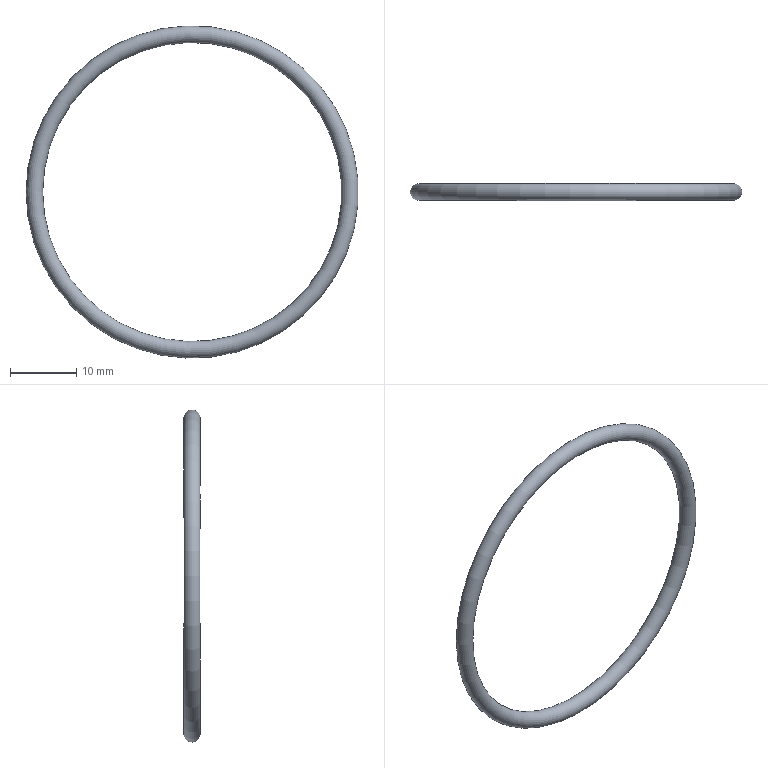Component | NX | O_RING | 1 solid | 1 faces | box 50 x 2.5 x 50 mm | volume 733 mm3 | torus 1
STEP:
#1=CARTESIAN_POINT('',(0.,0.,0.));
#2=DIRECTION('',(0.,0.,1.));
#3=DIRECTION('',(1.,0.,0.));
#4=AXIS2_PLACEMENT_3D('',#1,#2,#3);
#5=CARTESIAN_POINT('',(-25.,52.05,43.));
#6=VERTEX_POINT('',#5);
#7=CARTESIAN_POINT('',(-23.75,52.05,43.));
#8=DIRECTION('',(0.,0.,-1.));
#9=DIRECTION('',(-1.,0.,0.));
#10=AXIS2_PLACEMENT_3D('',#7,#8,#9);
#11=CIRCLE('',#10,1.25);
#12=CARTESIAN_POINT('',(-0.,52.05,43.));
#13=DIRECTION('',(0.,1.,0.));
#14=DIRECTION('',(-1.,0.,0.));
#15=AXIS2_PLACEMENT_3D('',#12,#13,#14);
#16=TOROIDAL_SURFACE('',#15,23.75,1.25);
#17=CARTESIAN_POINT('',(0.,0.));
#18=DIRECTION('',(0.,1.));
#19=VECTOR('',#18,1.);
#20=LINE('',#17,#19);
#21=(GEOMETRIC_REPRESENTATION_CONTEXT(2)PARAMETRIC_REPRESENTATION_CONTEXT()REPRESENTATION_CONTEXT('',''));
#22=DEFINITIONAL_REPRESENTATION('',(#20),#21);
#23=PCURVE('',#16,#22);
#24=CARTESIAN_POINT('',(6.283,0.));
#25=DIRECTION('',(0.,1.));
#26=VECTOR('',#25,1.);
#27=LINE('',#24,#26);
#28=(GEOMETRIC_REPRESENTATION_CONTEXT(2)PARAMETRIC_REPRESENTATION_CONTEXT()REPRESENTATION_CONTEXT('',''));
#29=DEFINITIONAL_REPRESENTATION('',(#27),#28);
#30=PCURVE('',#16,#29);
#31=SEAM_CURVE('',#11,(#23,#30),.PCURVE_S1.);
#32=EDGE_CURVE('',#6,#6,#31,.T.);
#33=ORIENTED_EDGE('',*,*,#32,.F.);
#34=CARTESIAN_POINT('',(-0.,52.05,43.));
#35=DIRECTION('',(0.,1.,0.));
#36=DIRECTION('',(-1.,0.,0.));
#37=AXIS2_PLACEMENT_3D('',#34,#35,#36);
#38=CIRCLE('',#37,25.);
#39=CARTESIAN_POINT('',(0.,0.));
#40=DIRECTION('',(1.,0.));
#41=VECTOR('',#40,1.);
#42=LINE('',#39,#41);
#43=(GEOMETRIC_REPRESENTATION_CONTEXT(2)PARAMETRIC_REPRESENTATION_CONTEXT()REPRESENTATION_CONTEXT('',''));
#44=DEFINITIONAL_REPRESENTATION('',(#42),#43);
#45=PCURVE('',#16,#44);
#46=CARTESIAN_POINT('',(0.,6.283));
#47=DIRECTION('',(1.,0.));
#48=VECTOR('',#47,1.);
#49=LINE('',#46,#48);
#50=(GEOMETRIC_REPRESENTATION_CONTEXT(2)PARAMETRIC_REPRESENTATION_CONTEXT()REPRESENTATION_CONTEXT('',''));
#51=DEFINITIONAL_REPRESENTATION('',(#49),#50);
#52=PCURVE('',#16,#51);
#53=SEAM_CURVE('',#38,(#45,#52),.PCURVE_S1.);
#54=EDGE_CURVE('',#6,#6,#53,.T.);
#55=ORIENTED_EDGE('',*,*,#54,.T.);
#56=ORIENTED_EDGE('',*,*,#32,.T.);
#57=ORIENTED_EDGE('',*,*,#54,.F.);
#58=EDGE_LOOP('',(#33,#55,#56,#57));
#59=FACE_BOUND('',#58,.T.);
#60=ADVANCED_FACE('',(#59),#16,.T.);
#61=CLOSED_SHELL('',(#60));
#62=MANIFOLD_SOLID_BREP('',#61);
#63=(LENGTH_UNIT()NAMED_UNIT(*)SI_UNIT(.MILLI.,.METRE.));
#64=UNCERTAINTY_MEASURE_WITH_UNIT(LENGTH_MEASURE(0.0000001),#63,'','');
#65=(NAMED_UNIT(*)PLANE_ANGLE_UNIT()SI_UNIT($,.RADIAN.));
#66=(NAMED_UNIT(*)SI_UNIT($,.STERADIAN.)SOLID_ANGLE_UNIT());
#67=(GEOMETRIC_REPRESENTATION_CONTEXT(3)GLOBAL_UNCERTAINTY_ASSIGNED_CONTEXT((#64))GLOBAL_UNIT_ASSIGNED_CONTEXT((#63,#65,#66))REPRESENTATION_CONTEXT('',''));
#68=ADVANCED_BREP_SHAPE_REPRESENTATION('',(#4,#62),#67);